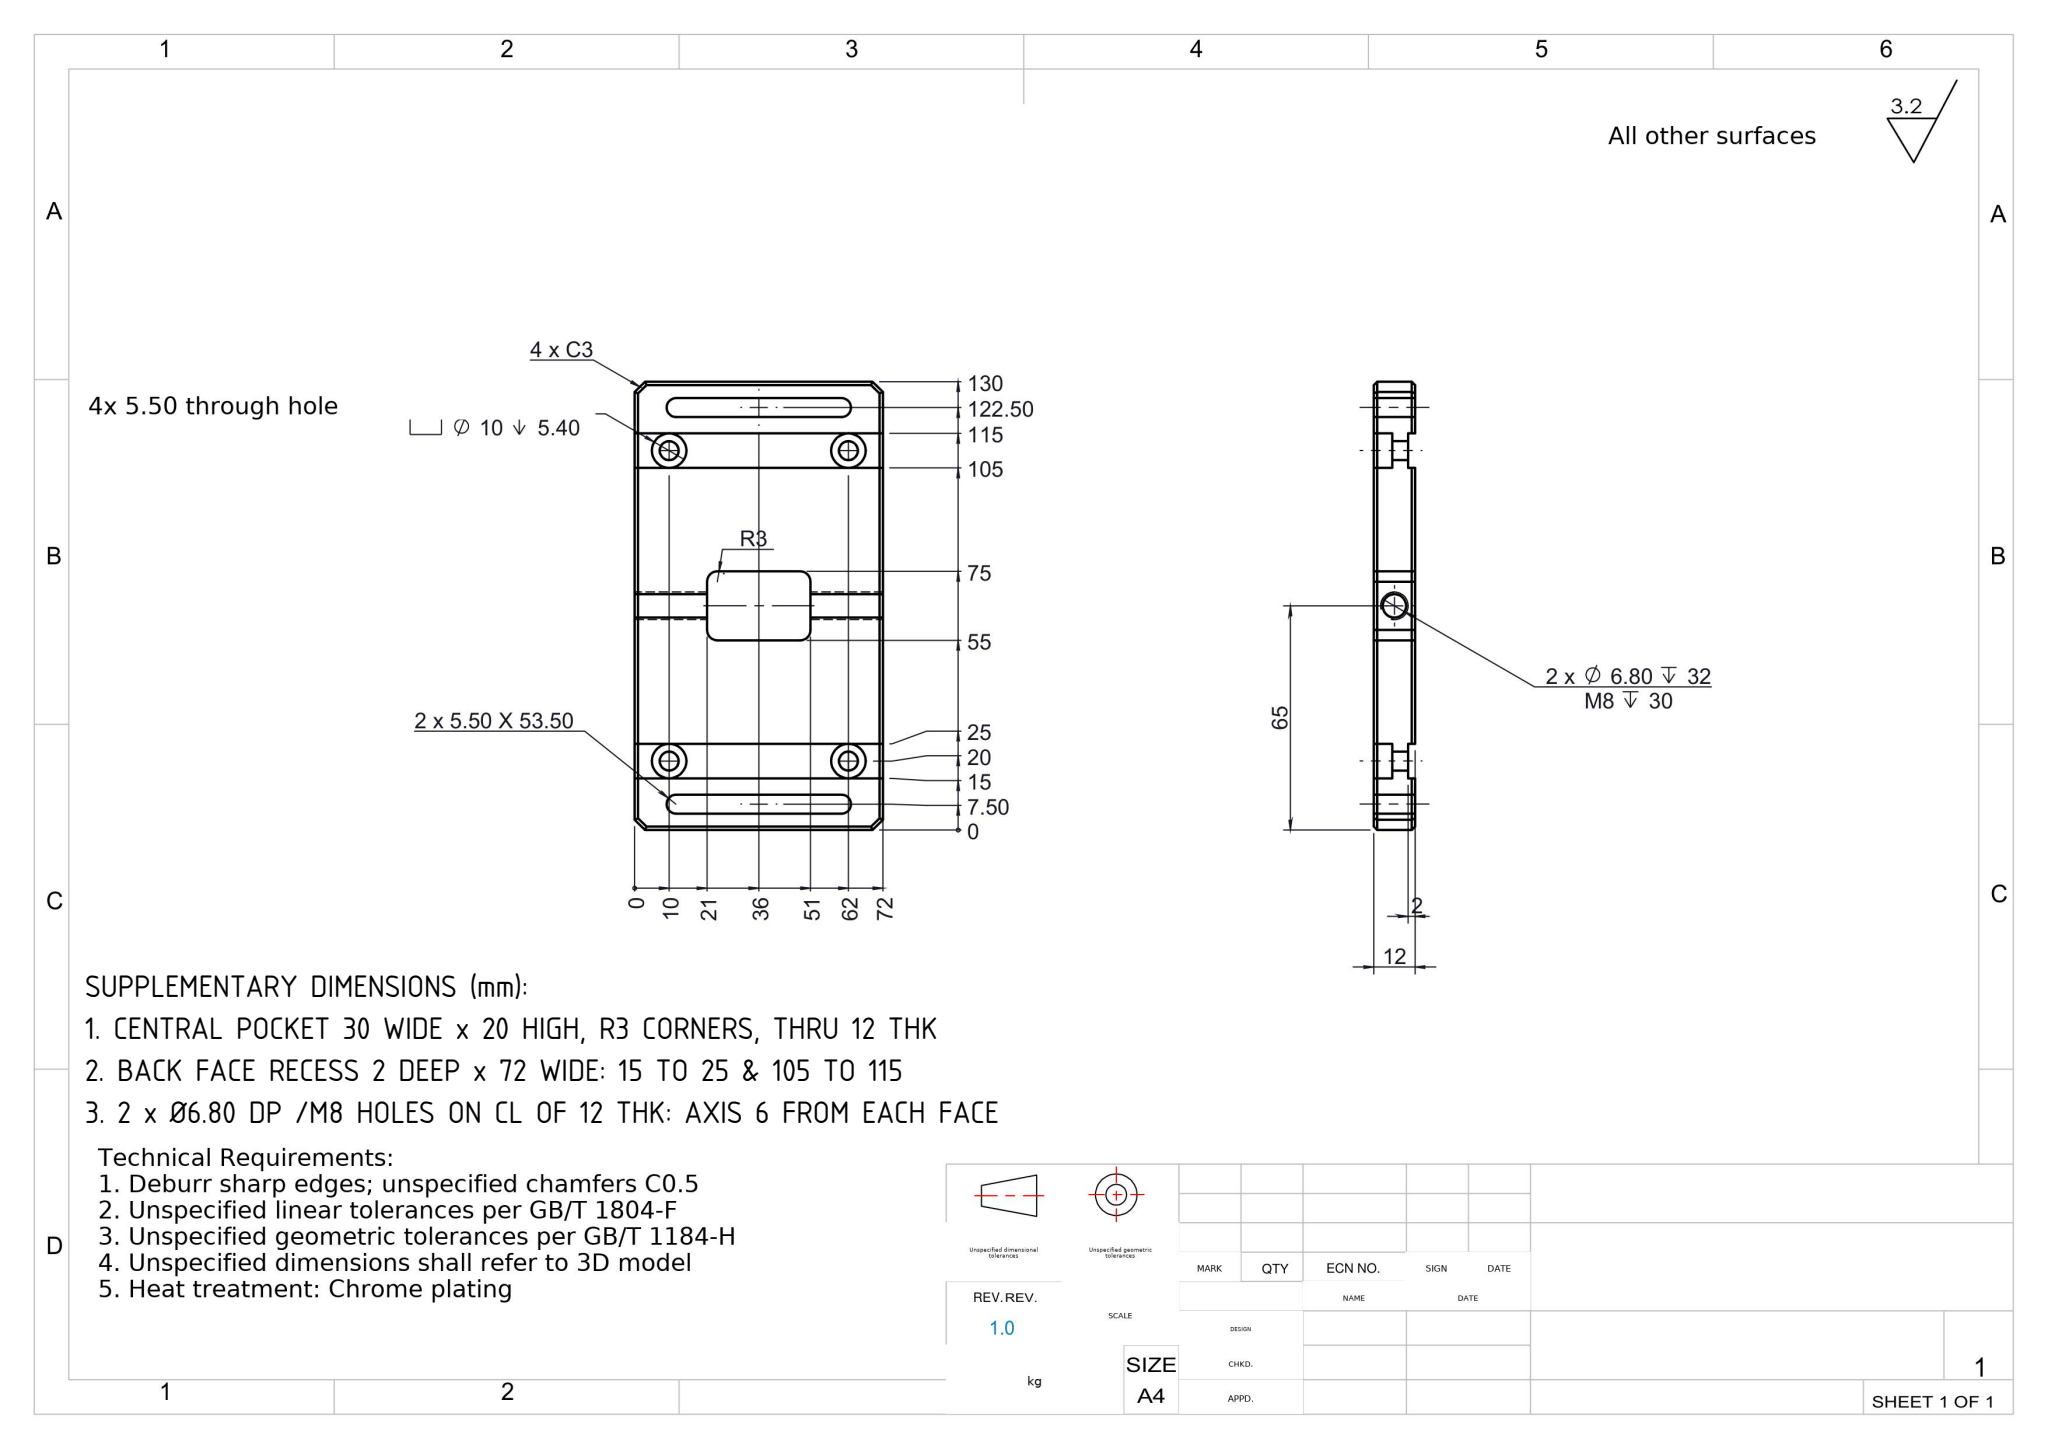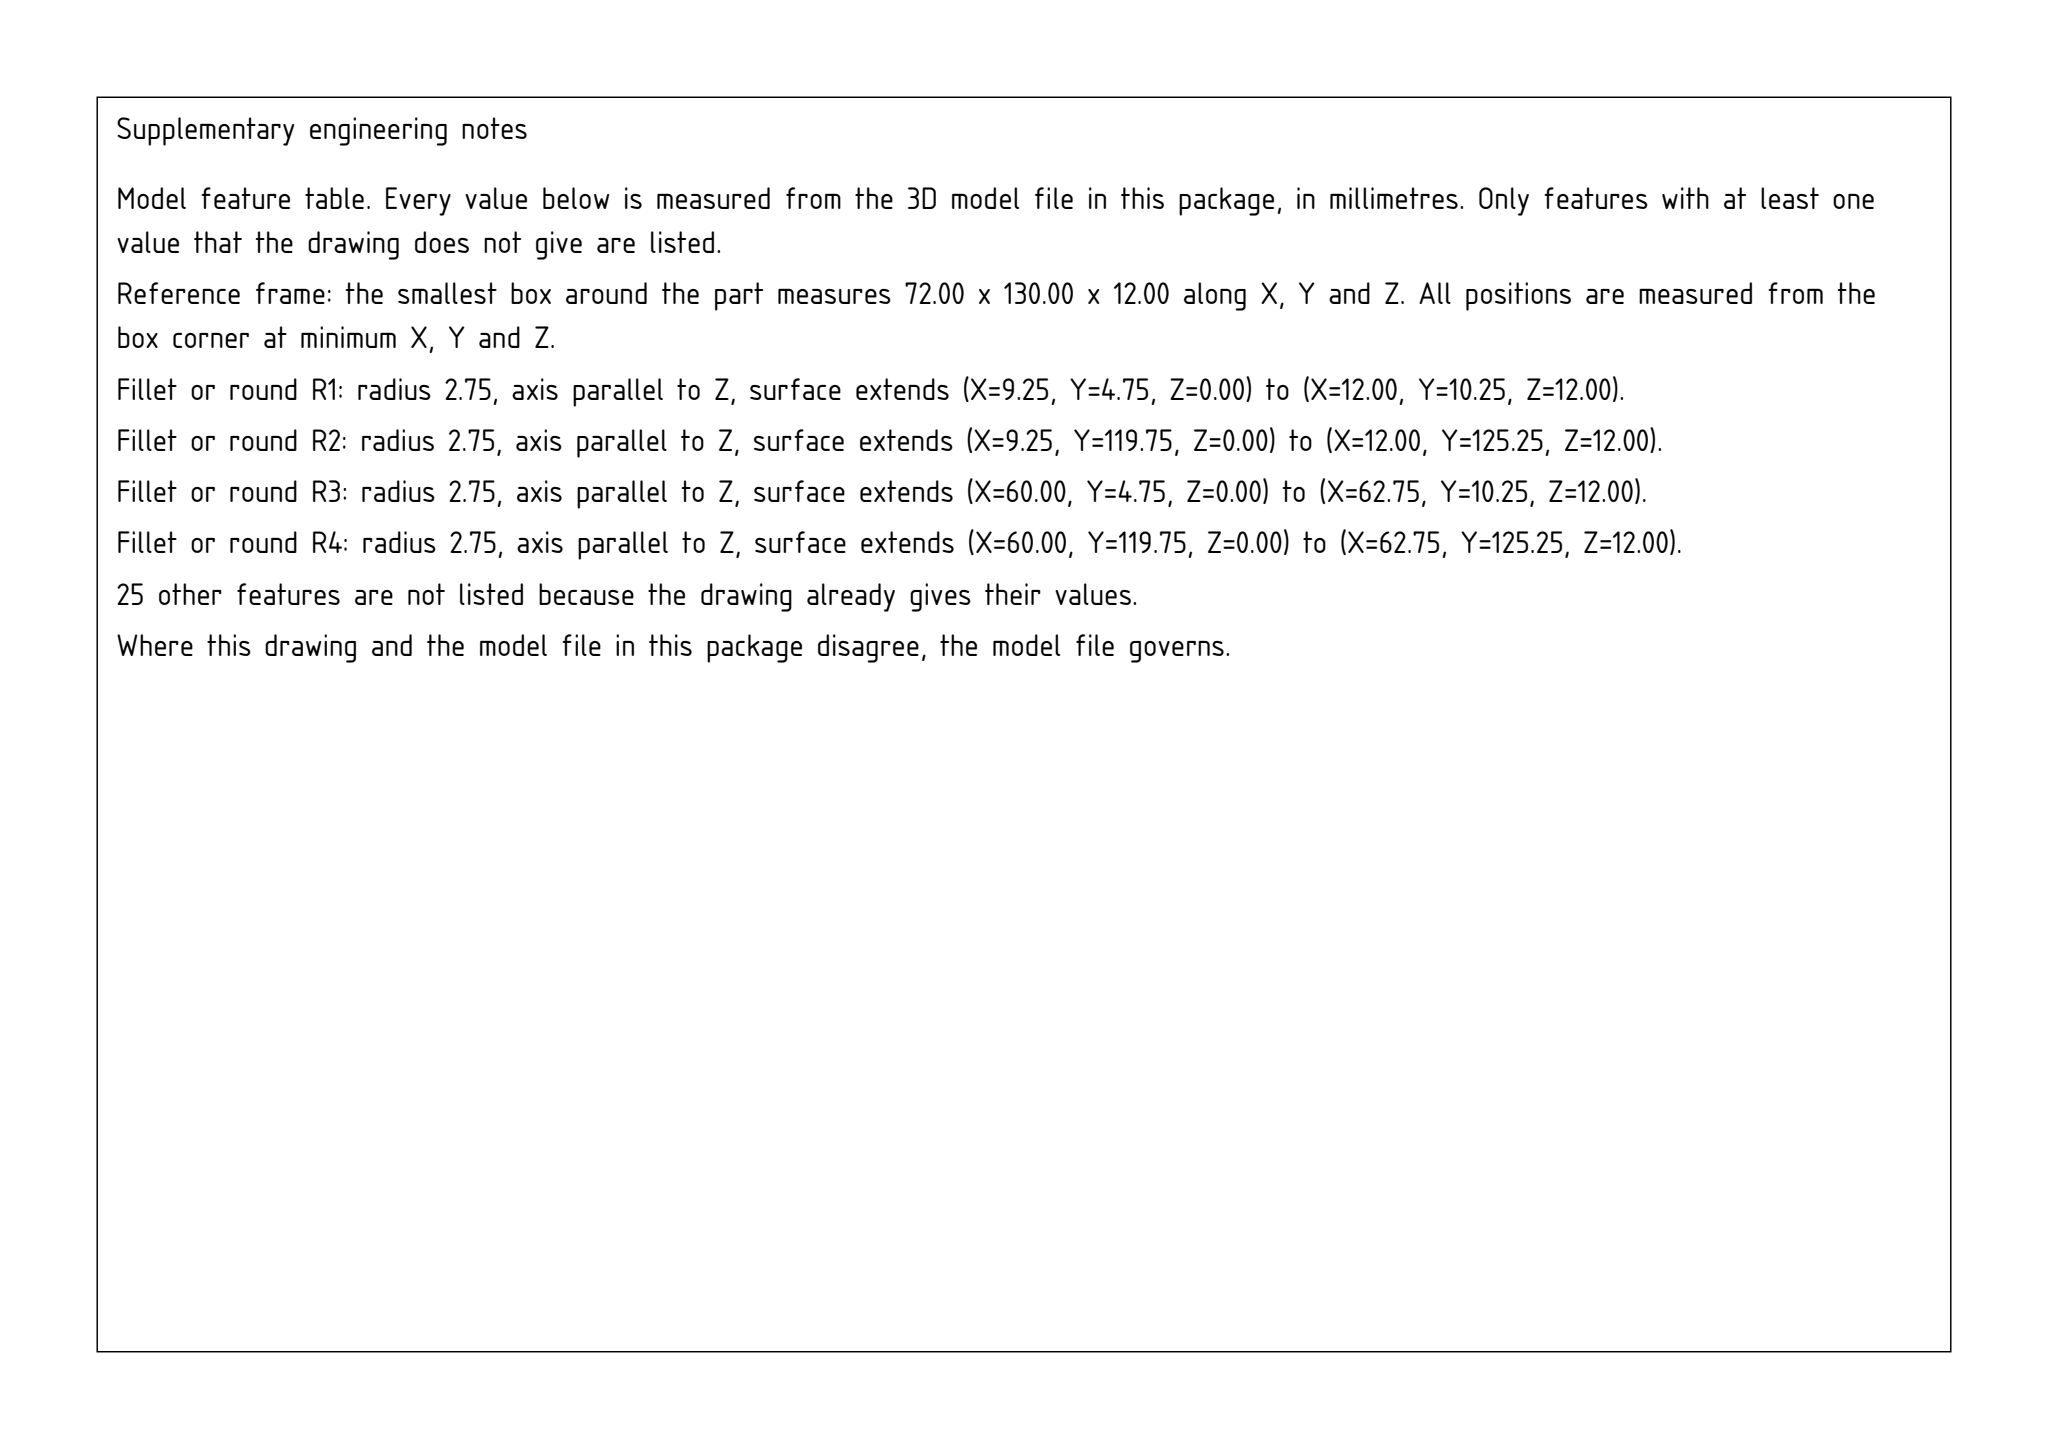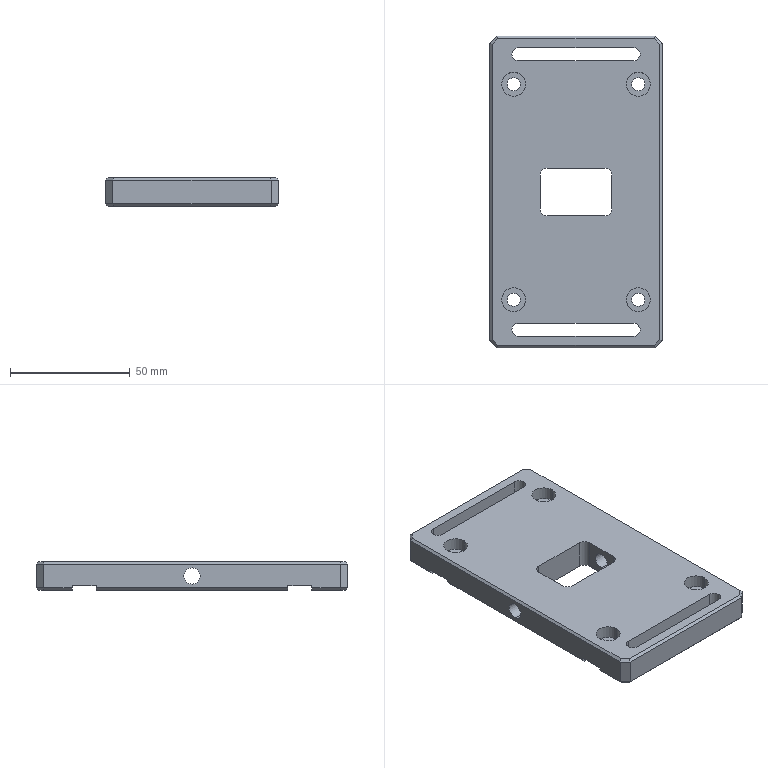Part | SolidWorks | mm | 1 solid | 80 faces | box 72 x 130 x 12 mm | volume 91177 mm3 | plane 50 | cylinder 30 | commonest cylinder face diameters 5.5 x14 10 x8 6.8 x4 6 x4
build123d program:
from build123d import *

# Parameters (mm, degrees)
SKETCH1_W                                       = 72
SKETCH1_H                                       = 130
BOSS_EXTRUDE1_DEPTH                             = 12
CHAMFER1_SIZE                                   = 3
CHAMFER2_SIZE                                   = 1
SKETCH2_W                                       = 2
SKETCH2_H                                       = 10
CUT_EXTRUDE1_DEPTH                              = 98.739
M5_HEX_SOCKET_HEAD_CAP_SCREW_CBORE1_D           = 5.5
M5_HEX_SOCKET_HEAD_CAP_SCREW_CBORE1_CBORE_D     = 10
M5_HEX_SOCKET_HEAD_CAP_SCREW_CBORE1_CBORE_DEPTH = 5.4
CUT_EXTRUDE2_DEPTH                              = 76.266
SKETCH9_W                                       = 30
SKETCH9_H                                       = 20
CUT_EXTRUDE3_DEPTH                              = 76.266
FILLET1_R                                       = 3


with BuildPart() as part:
    # Sketch1 → Boss-Extrude1 (new body)
    with BuildSketch(Plane.XY):
        Rectangle(SKETCH1_W, SKETCH1_H)
    extrude(amount=BOSS_EXTRUDE1_DEPTH)

    # Chamfer1
    chamfer1_edges = [part.edges().sort_by_distance(p)[0] for p in [
        (36, -65, 6),
        (-36, -65, 6),
        (-36, 65, 6),
        (36, 65, 6),
    ]]
    chamfer(chamfer1_edges, length=CHAMFER1_SIZE)

    # Chamfer2
    chamfer2_edges = [part.edges().sort_by_distance(p)[0] for p in [
        (-36, 0, 0),
        (-36, 0, 12),
        (36, 0, 0),
        (0, -65, 0),
        (0, 65, 0),
        (34.5, -63.5, 0),
        (-34.5, -63.5, 0),
        (34.5, 63.5, 0),
        (-34.5, 63.5, 0),
        (0, 65, 12),
        (36, 0, 12),
        (0, -65, 12),
        (34.5, -63.5, 12),
        (-34.5, -63.5, 12),
        (34.5, 63.5, 12),
        (-34.5, 63.5, 12),
    ]]
    chamfer(chamfer2_edges, length=CHAMFER2_SIZE)

    # Sketch2 → Cut-Extrude1 (cut, through all)
    with BuildSketch(Plane(origin=(36, 0, 0), x_dir=(0, 0, -1), z_dir=(1, 0, 0))):
        with Locations((-1, 45)):
            Rectangle(SKETCH2_W, SKETCH2_H)
        with Locations((-1, -45)):
            Rectangle(SKETCH2_W, SKETCH2_H)
    extrude(amount=-CUT_EXTRUDE1_DEPTH, mode=Mode.SUBTRACT)

    # M5 Hex Socket Head Cap Screw CBORE1 (through all)
    with Locations(Plane.XY.offset(12)):
        with Locations((26, -45), (-26, -45), (-26, 45), (26, 45)):
            CounterBoreHole(M5_HEX_SOCKET_HEAD_CAP_SCREW_CBORE1_D / 2, M5_HEX_SOCKET_HEAD_CAP_SCREW_CBORE1_CBORE_D / 2, M5_HEX_SOCKET_HEAD_CAP_SCREW_CBORE1_CBORE_DEPTH)

    # Sketch5 → Cut-Extrude2 (cut, through all)
    with BuildSketch(Plane(origin=(0, 0, 0), x_dir=(-1, 0, 0), z_dir=(0, 0, -1))):
        with BuildLine():
            Line((-24, 60.25), (24, 60.25))
            ThreePointArc((24, 60.25), (26.75, 57.5), (24, 54.75))
            Line((24, 54.75), (-24, 54.75))
            ThreePointArc((-24, 54.75), (-26.75, 57.5), (-24, 60.25))
        make_face()
        with BuildLine():
            Line((-24, -60.25), (24, -60.25))
            ThreePointArc((24, -60.25), (26.75, -57.5), (24, -54.75))
            Line((24, -54.75), (-24, -54.75))
            ThreePointArc((-24, -54.75), (-26.75, -57.5), (-24, -60.25))
        make_face()
    extrude(amount=-CUT_EXTRUDE2_DEPTH, mode=Mode.SUBTRACT)

    # Sketch7 → M8 Tapped Hole1 (revolve, cut)
    with BuildSketch(Plane(origin=(36, 0, 6), x_dir=(0, 0, -1), z_dir=(0, 1, 0))):
        Polygon((0, 0), (0, 34.043), (3.4, 32), (3.4, 0), align=None)
    m8_tapped_hole1 = revolve(axis=Axis((42.35, 0, 6), (-1, 0, 0)), mode=Mode.SUBTRACT)

    # Mirror1: M8 Tapped Hole1 across plane
    add(m8_tapped_hole1.mirror(Plane(origin=(0, 0, 0), x_dir=(0, 0, 1), z_dir=(1, 0, 0))), mode=Mode.SUBTRACT)

    # Sketch9 → Cut-Extrude3 (cut, through all)
    with BuildSketch(Plane(origin=(0, 0, 0), x_dir=(-1, 0, 0), z_dir=(0, 0, -1))):
        Rectangle(SKETCH9_W, SKETCH9_H)
    extrude(amount=-CUT_EXTRUDE3_DEPTH, mode=Mode.SUBTRACT)

    # Fillet1
    fillet1_edges = [part.edges().sort_by_distance(p)[0] for p in [
        (15, -10, 6),
        (-15, 10, 6),
        (-15, -10, 6),
        (15, 10, 6),
    ]]
    fillet(fillet1_edges, radius=FILLET1_R)


solid = part.part